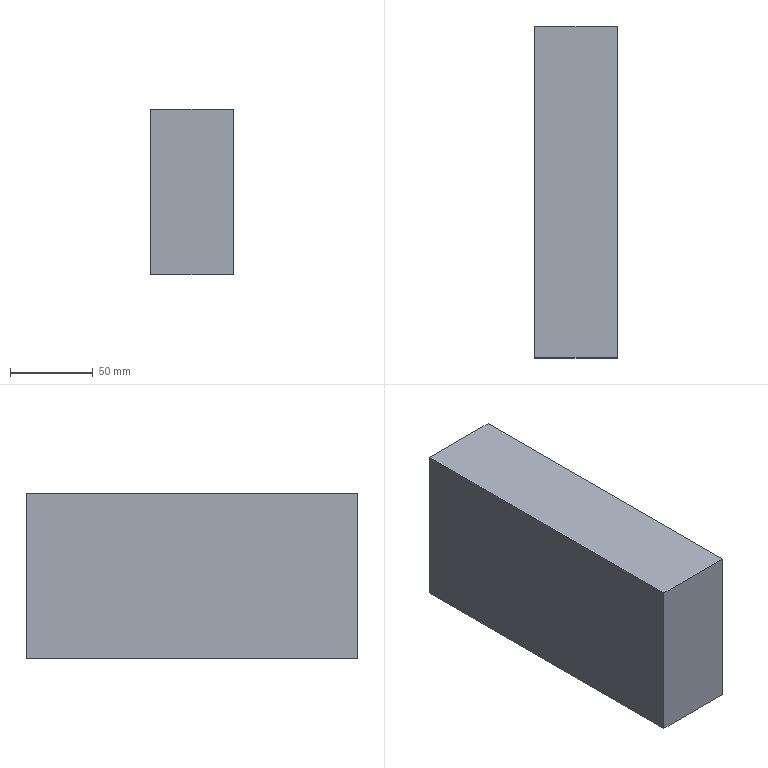Component | NX | GDLIANJIE_11 | 1 solid | 6 faces | volume 1000000 mm3 | plane 6